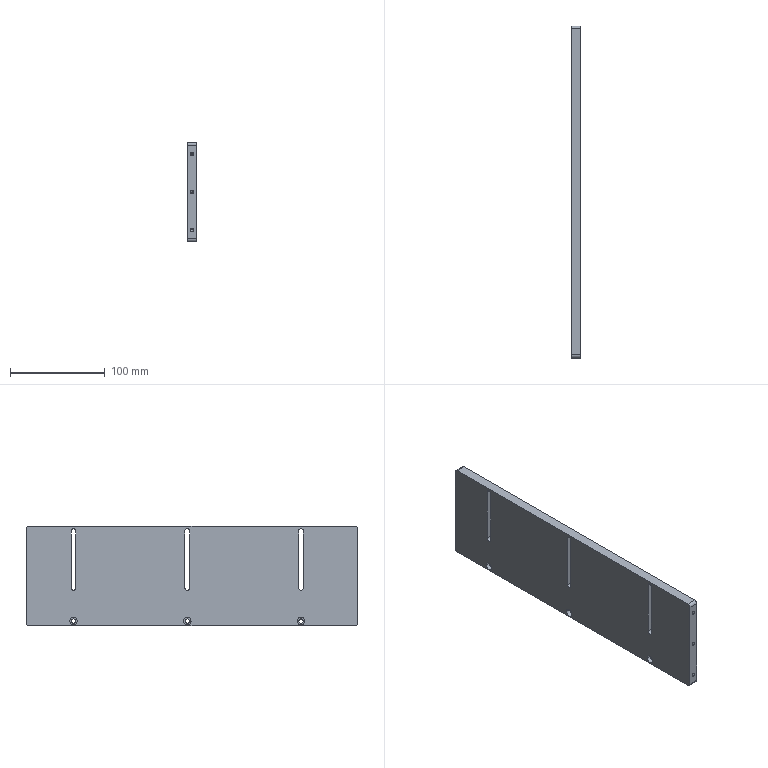Component | SolidWorks | SecondGenerationFour-sidedLabelingSideBaffle-1 | 1 solid | 49 faces | box 10 x 350 x 105 mm | volume 356435 mm3 | cylinder 28 | plane 15 | cone 6 | commonest cylinder face diameters 3.3 x6 8 x6 4.5 x6 5 x6 6 x4
build123d program:
from build123d import *

# Parameters (mm, degrees)
SKETCH1_W                                            = 105
SKETCH1_H                                            = 10
BOSS_EXTRUDE1_DEPTH                                  = 350
HOLE_SIZE_ACCORDING_TO_THE_TYPE_OF_HEXAG_D           = 4.5
HOLE_SIZE_ACCORDING_TO_THE_TYPE_OF_HEXAG_CBORE_D     = 8
HOLE_SIZE_ACCORDING_TO_THE_TYPE_OF_HEXAG_CBORE_DEPTH = 4.6
CUT_EXTRUDE1_DEPTH                                   = 355.057
M4_TAPPED_HOLE1_D                                    = 3.3
M4_TAPPED_HOLE1_DEPTH                                = 17.1
M4_TAPPED_HOLE1_TIP                                  = 0.9914
FILLET1_R                                            = 3


with BuildPart() as part:
    # Sketch1 → Boss-Extrude1 (new body)
    with BuildSketch(Plane.XY):
        Rectangle(SKETCH1_W, SKETCH1_H)
    extrude(amount=BOSS_EXTRUDE1_DEPTH)

    # Hole Size according to the type of Hexag (through all)
    with Locations(Plane(origin=(0, 5, 0), x_dir=(-1, 0, 0), z_dir=(0, 1, 0))):
        with Locations((-47.5, 180), (-47.5, 300), (-47.5, 60)):
            CounterBoreHole(HOLE_SIZE_ACCORDING_TO_THE_TYPE_OF_HEXAG_D / 2, HOLE_SIZE_ACCORDING_TO_THE_TYPE_OF_HEXAG_CBORE_D / 2, HOLE_SIZE_ACCORDING_TO_THE_TYPE_OF_HEXAG_CBORE_DEPTH)

    # Sketch4 → Cut-Extrude1 (cut, through all)
    with BuildSketch(Plane(origin=(0, 5, 0), x_dir=(1, 0, 0), z_dir=(0, 1, 0))):
        with BuildLine():
            Line((-47.5, -57.5), (12.5, -57.5))
            ThreePointArc((12.5, -57.5), (15, -60), (12.5, -62.5))
            Line((12.5, -62.5), (-47.5, -62.5))
            ThreePointArc((-47.5, -62.5), (-50, -60), (-47.5, -57.5))
        make_face()
        with BuildLine():
            Line((-47.5, -297.5), (12.5, -297.5))
            ThreePointArc((12.5, -297.5), (15, -300), (12.5, -302.5))
            Line((12.5, -302.5), (-47.5, -302.5))
            ThreePointArc((-47.5, -302.5), (-50, -300), (-47.5, -297.5))
        make_face()
        with BuildLine():
            Line((-47.5, -177.5), (12.5, -177.5))
            ThreePointArc((12.5, -177.5), (15, -180), (12.5, -182.5))
            Line((12.5, -182.5), (-47.5, -182.5))
            ThreePointArc((-47.5, -182.5), (-50, -180), (-47.5, -177.5))
        make_face()
    extrude(amount=-CUT_EXTRUDE1_DEPTH, mode=Mode.SUBTRACT)

    # M4 Tapped Hole1
    with Locations(Plane(origin=(0, 0, 0), x_dir=(-1, 0, 0), z_dir=(0, 0, -1))):
        with Locations((-40, 0), (40, 0), (0, 0)):
            Hole(M4_TAPPED_HOLE1_D / 2, depth=M4_TAPPED_HOLE1_DEPTH)
            with Locations((0, 0, -(M4_TAPPED_HOLE1_DEPTH + M4_TAPPED_HOLE1_TIP / 2))):  # 118° drill point
                Cone(0, M4_TAPPED_HOLE1_D / 2, M4_TAPPED_HOLE1_TIP, mode=Mode.SUBTRACT)

    # Fillet1
    fillet1_edges = [part.edges().sort_by_distance(p)[0] for p in [
        (52.5, 0, 350),
        (-52.5, 0, 350),
        (52.5, 0, 0),
        (-52.5, 0, 0),
    ]]
    fillet(fillet1_edges, radius=FILLET1_R)


solid = part.part

# Placed as in the assembly
solid = solid.moved(Location((-75.027, 41.863, -71.5), (-90, 0, 90)))